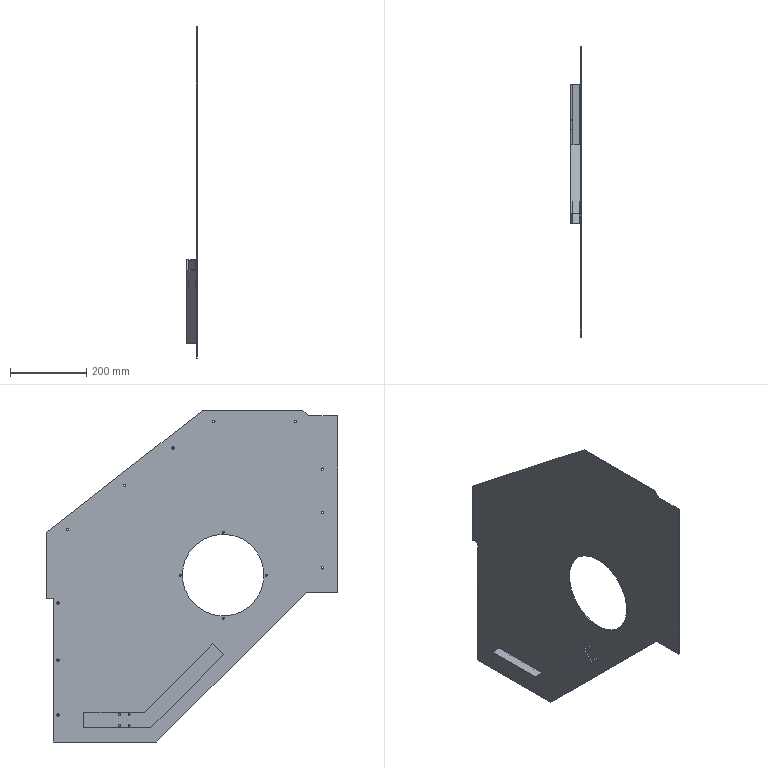Component | SolidWorks | MiddleBaffle-1 | 2 solids | 71 faces | box 27 x 764.98 x 872.71 mm | volume 1046797 mm3 | cylinder 40 | plane 31 | commonest cylinder face diameters 6 x22 5.2 x16 215 x2
build123d program:
from build123d import *

# Parameters (mm, degrees)
BOSS_EXTRUDE1_2_DEPTH    = 2
SKETCH2_R                = 107.5
CUT_EXTRUDE1_DEPTH       = 2
SKETCH5_R                = 3
CUT_EXTRUDE3_DEPTH       = 2
SKETCH6_R                = 3
CUT_EXTRUDE4_DEPTH       = 2
BOSS_EXTRUDE2_DEPTH      = 25
SHELL1_T                 = -3
SKETCH8_R                = 2.6
CUT_EXTRUDE5_DEPTH       = 2
SKETCH9_R                = 2.6
CUT_EXTRUDE6_DEPTH       = 2
BOSS_EXTRUDE1_DEPTH      = 3
BOSS_EXTRUDE1_DEPTH_BACK = 1
SKETCH1_W                = 13.752
SKETCH1_H                = 33.192


with BuildPart() as part:
    # Sketch1_2 → Boss-Extrude1_2 (new body)
    with BuildSketch(Plane.XY):
        Polygon((-144.8, -39.078), (-144.8, 222.922), (177, 634.808), (359.25, 634.808), (359.25, 616.808), (727.912, 616.808), (727.912, 344.609), (335.468, -47.835), (335.468, -130.175), (-129.802, -130.175), (-129.802, -54.075), align=None)
    extrude(amount=BOSS_EXTRUDE1_2_DEPTH)

    # Sketch2 → Cut-Extrude1 (cut)
    with BuildSketch(Plane.XY.offset(2)):
        with Locations((289.2, 170.355)):
            Circle(SKETCH2_R)
    extrude(amount=-CUT_EXTRUDE1_DEPTH, mode=Mode.SUBTRACT)

    # Sketch5 → Cut-Extrude3 (cut)
    with BuildSketch(Plane(origin=(0, 0, 0), x_dir=(-1, 0, 0), z_dir=(0, 0, -1))):
        with Locations((114.8, -20.176)):
            Circle(SKETCH5_R)
        with Locations((114.8, 194.824)):
            Circle(SKETCH5_R)
        with Locations((44.88, 302.102)):
            Circle(SKETCH5_R)
        with Locations((-52.737, 428.874)):
            Circle(SKETCH5_R)
        with Locations((-168.532, 579.511)):
            Circle(SKETCH5_R)
        with Locations((-362.247, 604.825)):
            Circle(SKETCH5_R)
        with Locations((-512.649, 604.808)):
            Circle(SKETCH5_R)
        with Locations((-657.182, 604.808)):
            Circle(SKETCH5_R)
    extrude(amount=-CUT_EXTRUDE3_DEPTH, mode=Mode.SUBTRACT)

    # Sketch6 → Cut-Extrude4 (cut)
    with BuildSketch(Plane.XY.offset(2)):
        with Locations((270.468, -90.175)):
            Circle(SKETCH6_R)
        with Locations((125.468, -90.175)):
            Circle(SKETCH6_R)
        with Locations((10.468, -90.175)):
            Circle(SKETCH6_R)
    extrude(amount=-CUT_EXTRUDE4_DEPTH, mode=Mode.SUBTRACT)

    # Sketch8 → Cut-Extrude5 (cut)
    with BuildSketch(Plane.XY.offset(2)):
        with Locations((289.2, 283.355)):
            Circle(SKETCH8_R)
        with Locations((402.2, 170.355)):
            Circle(SKETCH8_R)
        with Locations((289.2, 57.355)):
            Circle(SKETCH8_R)
        with Locations((176.2, 170.355)):
            Circle(SKETCH8_R)
    extrude(amount=-CUT_EXTRUDE5_DEPTH, mode=Mode.SUBTRACT)


with BuildPart() as body_2:
    # Sketch7 → Boss-Extrude2 (new body)
    with BuildSketch(Plane(origin=(0, 0, 0), x_dir=(-1, 0, 0), z_dir=(0, 0, -1))):
        Polygon((-689.912, 536.808), (-649.912, 536.808), (-649.912, 376.918), (-470.269, 197.274), (-498.553, 168.99), (-689.912, 360.349), align=None)
    extrude(amount=BOSS_EXTRUDE2_DEPTH)

    # Shell1
    shell1_openings = [body_2.faces().sort_by_distance(p)[0] for p in [
        (669.912, 536.808, -12.5),
        (484.411, 183.132, -12.5),
    ]]
    offset(amount=SHELL1_T, openings=shell1_openings, kind=Kind.INTERSECTION)

    # Sketch9 → Cut-Extrude6 (cut)
    with BuildSketch(Plane(origin=(0, 0, -25), x_dir=(-1, 0, 0), z_dir=(0, 0, -1))):
        with Locations((-683.912, 442.825)):
            Circle(SKETCH9_R)
        with Locations((-655.912, 442.825)):
            Circle(SKETCH9_R)
        with Locations((-655.912, 417.825)):
            Circle(SKETCH9_R)
        with Locations((-683.912, 417.825)):
            Circle(SKETCH9_R)
    extrude(amount=-CUT_EXTRUDE6_DEPTH, mode=Mode.SUBTRACT)


with BuildPart() as body_3:
    # Sketch1 → Boss-Extrude1 (new, two sides: drawn at the far end of the back side and taken through both)
    with BuildSketch(Plane.XY.offset(-BOSS_EXTRUDE1_DEPTH_BACK)):
        with Locations((358.124, 633.404)):
            Rectangle(SKETCH1_W, SKETCH1_H)
    extrude(amount=BOSS_EXTRUDE1_DEPTH + BOSS_EXTRUDE1_DEPTH_BACK)


with BuildPart() as part_1:
    add(part.part)

    # Door Rear Lip Clearance Cutout: cut body 3
    add(body_3.part, mode=Mode.SUBTRACT)


solid = Compound([body_2.part, part_1.part])

# Placed as in the assembly
solid = solid.moved(Location((-294.55, -248.256, 346.681), (0, 90, 0)))